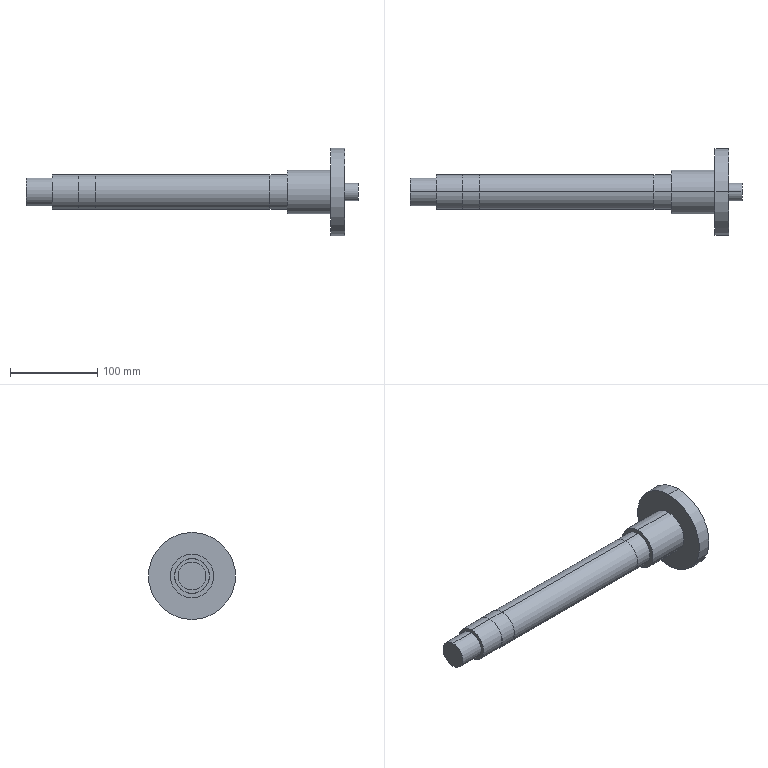Component | SolidWorks | Axis-1 | 1 solid | 25 faces | box 381 x 100 x 100 mm | volume 589087 mm3 | cylinder 16 | plane 9 | commonest cylinder face diameters 39.8 x4 40 x4 20 x2 32 x2 100 x2 50 x2
build123d program:
from build123d import *

# Parameters (mm, degrees)
SKETCH2_OUTSIDE_W   = 180.474
SKETCH2_OUTSIDE_H   = 180.474
SKETCH2_OUTSIDE_R   = 19.9
CUT_EXTRUDE1_DEPTH  = 30
SKETCH3_R           = 10
BOSS_EXTRUDE1_DEPTH = 15


with BuildPart() as part:
    # Sketch1 → Revolve1 (revolve)
    with BuildSketch(Plane.XY, mode=Mode.PRIVATE) as revolve1_sk:
        Polygon((0, 0), (0, 16), (30, 16), (30, 20), (80, 20), (80, 19.9), (280, 19.9), (280, 20), (300, 20), (300, 25), (350, 25), (350, 50), (366, 50), (366, 0), align=None)
    revolve(revolve1_sk.sketch.rotate(Axis((-164.625, 0, 0), (1, 0, 0)), 90), axis=Axis((-164.625, 0, 0), (1, 0, 0)))

    # Sketch2 outside → Cut-Extrude1 (cut)
    with BuildSketch(Plane.ZY.offset(-30)):
        Rectangle(SKETCH2_OUTSIDE_W, SKETCH2_OUTSIDE_H)
        Circle(SKETCH2_OUTSIDE_R, mode=Mode.SUBTRACT)
    extrude(amount=-CUT_EXTRUDE1_DEPTH, mode=Mode.SUBTRACT)

    # Sketch3 → Boss-Extrude1 (add)
    with BuildSketch(Plane(origin=(366, 0, 0), x_dir=(0, 0, -1), z_dir=(1, 0, 0))):
        with Locations(Location((0, 0, 0), (0, 0, 180))):
            Circle(SKETCH3_R)
    extrude(amount=BOSS_EXTRUDE1_DEPTH)


solid = part.part

# Placed as in the assembly
solid = solid.moved(Location((-372.743, 1299.706, 687.116), (0, 0, 0)))
STEP:
#1=COLOUR_RGB('',0.7922,0.8196,0.9333);
#2=FILL_AREA_STYLE_COLOUR('',#1);
#3=FILL_AREA_STYLE('',(#2));
#4=SURFACE_STYLE_FILL_AREA(#3);
#5=SURFACE_SIDE_STYLE('',(#4));
#6=SURFACE_STYLE_USAGE(.BOTH.,#5);
#7=PRESENTATION_STYLE_ASSIGNMENT((#6));
#8=CARTESIAN_POINT('',(0.3251,51.17,26.658));
#9=VERTEX_POINT('',#8);
#10=CARTESIAN_POINT('',(0.3251,51.17,27.446));
#11=VERTEX_POINT('',#10);
#12=CARTESIAN_POINT('',(0.3251,51.17,27.052));
#13=DIRECTION('',(1.,0.,0.));
#14=DIRECTION('',(0.,0.,-1.));
#15=AXIS2_PLACEMENT_3D('',#12,#13,#14);
#16=CIRCLE('',#15,0.3937);
#17=EDGE_CURVE('',#9,#11,#16,.T.);
#18=ORIENTED_EDGE('',*,*,#17,.F.);
#19=CARTESIAN_POINT('',(-0.2655,51.17,26.658));
#20=VERTEX_POINT('',#19);
#21=CARTESIAN_POINT('',(0.3251,51.17,26.658));
#22=DIRECTION('',(-1.,0.,0.));
#23=VECTOR('',#22,39.37);
#24=LINE('',#21,#23);
#25=EDGE_CURVE('',#9,#20,#24,.T.);
#26=ORIENTED_EDGE('',*,*,#25,.T.);
#27=CARTESIAN_POINT('',(-0.2655,51.17,27.446));
#28=VERTEX_POINT('',#27);
#29=CARTESIAN_POINT('',(-0.2655,51.17,27.052));
#30=DIRECTION('',(1.,0.,0.));
#31=DIRECTION('',(0.,0.,1.));
#32=AXIS2_PLACEMENT_3D('',#29,#30,#31);
#33=CIRCLE('',#32,0.3937);
#34=EDGE_CURVE('',#20,#28,#33,.T.);
#35=ORIENTED_EDGE('',*,*,#34,.T.);
#36=CARTESIAN_POINT('',(0.3251,51.17,27.446));
#37=DIRECTION('',(-1.,0.,0.));
#38=VECTOR('',#37,39.37);
#39=LINE('',#36,#38);
#40=EDGE_CURVE('',#11,#28,#39,.T.);
#41=ORIENTED_EDGE('',*,*,#40,.F.);
#42=EDGE_LOOP('',(#18,#26,#35,#41));
#43=FACE_OUTER_BOUND('',#42,.T.);
#44=CARTESIAN_POINT('',(0.3251,51.17,27.052));
#45=DIRECTION('',(-1.,0.,0.));
#46=DIRECTION('',(0.,0.,1.));
#47=AXIS2_PLACEMENT_3D('',#44,#45,#46);
#48=CYLINDRICAL_SURFACE('',#47,0.3937);
#49=ADVANCED_FACE('',(#43),#48,.T.);
#50=CARTESIAN_POINT('',(-13.494,51.17,27.682));
#51=VERTEX_POINT('',#50);
#52=CARTESIAN_POINT('',(-13.494,51.17,26.422));
#53=VERTEX_POINT('',#52);
#54=CARTESIAN_POINT('',(-13.494,51.17,27.052));
#55=DIRECTION('',(-1.,0.,0.));
#56=DIRECTION('',(0.,0.,1.));
#57=AXIS2_PLACEMENT_3D('',#54,#55,#56);
#58=CIRCLE('',#57,0.6299);
#59=EDGE_CURVE('',#51,#53,#58,.T.);
#60=ORIENTED_EDGE('',*,*,#59,.T.);
#61=CARTESIAN_POINT('',(-14.675,51.17,26.422));
#62=VERTEX_POINT('',#61);
#63=CARTESIAN_POINT('',(-21.156,51.17,26.422));
#64=DIRECTION('',(-1.,0.,0.));
#65=VECTOR('',#64,39.37);
#66=LINE('',#63,#65);
#67=EDGE_CURVE('',#53,#62,#66,.T.);
#68=ORIENTED_EDGE('',*,*,#67,.T.);
#69=CARTESIAN_POINT('',(-14.675,51.17,27.682));
#70=VERTEX_POINT('',#69);
#71=CARTESIAN_POINT('',(-14.675,51.17,27.052));
#72=DIRECTION('',(-1.,0.,0.));
#73=DIRECTION('',(0.,0.,1.));
#74=AXIS2_PLACEMENT_3D('',#71,#72,#73);
#75=CIRCLE('',#74,0.6299);
#76=EDGE_CURVE('',#70,#62,#75,.T.);
#77=ORIENTED_EDGE('',*,*,#76,.F.);
#78=CARTESIAN_POINT('',(-21.156,51.17,27.682));
#79=DIRECTION('',(-1.,0.,0.));
#80=VECTOR('',#79,39.37);
#81=LINE('',#78,#80);
#82=EDGE_CURVE('',#51,#70,#81,.T.);
#83=ORIENTED_EDGE('',*,*,#82,.F.);
#84=EDGE_LOOP('',(#60,#68,#77,#83));
#85=FACE_OUTER_BOUND('',#84,.T.);
#86=CARTESIAN_POINT('',(-21.156,51.17,27.052));
#87=DIRECTION('',(-1.,0.,0.));
#88=DIRECTION('',(0.,0.,1.));
#89=AXIS2_PLACEMENT_3D('',#86,#87,#88);
#90=CYLINDRICAL_SURFACE('',#89,0.6299);
#91=ADVANCED_FACE('',(#85),#90,.T.);
#92=CARTESIAN_POINT('',(-12.313,51.17,27.835));
#93=VERTEX_POINT('',#92);
#94=CARTESIAN_POINT('',(-12.313,51.17,26.268));
#95=VERTEX_POINT('',#94);
#96=CARTESIAN_POINT('',(-12.313,51.17,27.052));
#97=DIRECTION('',(-1.,0.,0.));
#98=DIRECTION('',(0.,0.,1.));
#99=AXIS2_PLACEMENT_3D('',#96,#97,#98);
#100=CIRCLE('',#99,0.7835);
#101=EDGE_CURVE('',#93,#95,#100,.T.);
#102=ORIENTED_EDGE('',*,*,#101,.T.);
#103=CARTESIAN_POINT('',(-13.494,51.17,26.268));
#104=VERTEX_POINT('',#103);
#105=CARTESIAN_POINT('',(-12.313,51.17,26.268));
#106=DIRECTION('',(-1.,0.,0.));
#107=VECTOR('',#106,39.37);
#108=LINE('',#105,#107);
#109=EDGE_CURVE('',#95,#104,#108,.T.);
#110=ORIENTED_EDGE('',*,*,#109,.T.);
#111=CARTESIAN_POINT('',(-13.494,51.17,27.835));
#112=VERTEX_POINT('',#111);
#113=CARTESIAN_POINT('',(-13.494,51.17,27.052));
#114=DIRECTION('',(-1.,0.,0.));
#115=DIRECTION('',(0.,0.,1.));
#116=AXIS2_PLACEMENT_3D('',#113,#114,#115);
#117=CIRCLE('',#116,0.7835);
#118=EDGE_CURVE('',#112,#104,#117,.T.);
#119=ORIENTED_EDGE('',*,*,#118,.F.);
#120=CARTESIAN_POINT('',(-12.313,51.17,27.835));
#121=DIRECTION('',(-1.,0.,0.));
#122=VECTOR('',#121,39.37);
#123=LINE('',#120,#122);
#124=EDGE_CURVE('',#93,#112,#123,.T.);
#125=ORIENTED_EDGE('',*,*,#124,.F.);
#126=EDGE_LOOP('',(#102,#110,#119,#125));
#127=FACE_OUTER_BOUND('',#126,.T.);
#128=CARTESIAN_POINT('',(-12.313,51.17,27.052));
#129=DIRECTION('',(-1.,0.,0.));
#130=DIRECTION('',(0.,0.,1.));
#131=AXIS2_PLACEMENT_3D('',#128,#129,#130);
#132=CYLINDRICAL_SURFACE('',#131,0.7835);
#133=ADVANCED_FACE('',(#127),#132,.T.);
#134=CARTESIAN_POINT('',(-0.2655,51.17,29.02));
#135=VERTEX_POINT('',#134);
#136=CARTESIAN_POINT('',(-0.2655,51.17,25.083));
#137=VERTEX_POINT('',#136);
#138=CARTESIAN_POINT('',(-0.2655,51.17,27.052));
#139=DIRECTION('',(-1.,0.,0.));
#140=DIRECTION('',(0.,0.,1.));
#141=AXIS2_PLACEMENT_3D('',#138,#139,#140);
#142=CIRCLE('',#141,1.969);
#143=EDGE_CURVE('',#135,#137,#142,.T.);
#144=ORIENTED_EDGE('',*,*,#143,.T.);
#145=CARTESIAN_POINT('',(-0.8954,51.17,25.083));
#146=VERTEX_POINT('',#145);
#147=CARTESIAN_POINT('',(-21.156,51.17,25.083));
#148=DIRECTION('',(-1.,0.,0.));
#149=VECTOR('',#148,39.37);
#150=LINE('',#147,#149);
#151=EDGE_CURVE('',#137,#146,#150,.T.);
#152=ORIENTED_EDGE('',*,*,#151,.T.);
#153=CARTESIAN_POINT('',(-0.8954,51.17,29.02));
#154=VERTEX_POINT('',#153);
#155=CARTESIAN_POINT('',(-0.8954,51.17,27.052));
#156=DIRECTION('',(-1.,0.,0.));
#157=DIRECTION('',(0.,0.,1.));
#158=AXIS2_PLACEMENT_3D('',#155,#156,#157);
#159=CIRCLE('',#158,1.969);
#160=EDGE_CURVE('',#154,#146,#159,.T.);
#161=ORIENTED_EDGE('',*,*,#160,.F.);
#162=CARTESIAN_POINT('',(-21.156,51.17,29.02));
#163=DIRECTION('',(-1.,0.,0.));
#164=VECTOR('',#163,39.37);
#165=LINE('',#162,#164);
#166=EDGE_CURVE('',#135,#154,#165,.T.);
#167=ORIENTED_EDGE('',*,*,#166,.F.);
#168=EDGE_LOOP('',(#144,#152,#161,#167));
#169=FACE_OUTER_BOUND('',#168,.T.);
#170=CARTESIAN_POINT('',(-21.156,51.17,27.052));
#171=DIRECTION('',(-1.,0.,0.));
#172=DIRECTION('',(0.,0.,1.));
#173=AXIS2_PLACEMENT_3D('',#170,#171,#172);
#174=CYLINDRICAL_SURFACE('',#173,1.969);
#175=ADVANCED_FACE('',(#169),#174,.T.);
#176=CARTESIAN_POINT('',(-0.8954,51.17,28.036));
#177=VERTEX_POINT('',#176);
#178=CARTESIAN_POINT('',(-0.8954,51.17,26.068));
#179=VERTEX_POINT('',#178);
#180=CARTESIAN_POINT('',(-0.8954,51.17,27.052));
#181=DIRECTION('',(-1.,0.,0.));
#182=DIRECTION('',(0.,0.,1.));
#183=AXIS2_PLACEMENT_3D('',#180,#181,#182);
#184=CIRCLE('',#183,0.9843);
#185=EDGE_CURVE('',#177,#179,#184,.T.);
#186=ORIENTED_EDGE('',*,*,#185,.T.);
#187=CARTESIAN_POINT('',(-2.864,51.17,26.068));
#188=VERTEX_POINT('',#187);
#189=CARTESIAN_POINT('',(-21.156,51.17,26.068));
#190=DIRECTION('',(-1.,0.,0.));
#191=VECTOR('',#190,39.37);
#192=LINE('',#189,#191);
#193=EDGE_CURVE('',#179,#188,#192,.T.);
#194=ORIENTED_EDGE('',*,*,#193,.T.);
#195=CARTESIAN_POINT('',(-2.864,51.17,28.036));
#196=VERTEX_POINT('',#195);
#197=CARTESIAN_POINT('',(-2.864,51.17,27.052));
#198=DIRECTION('',(-1.,0.,0.));
#199=DIRECTION('',(0.,0.,1.));
#200=AXIS2_PLACEMENT_3D('',#197,#198,#199);
#201=CIRCLE('',#200,0.9843);
#202=EDGE_CURVE('',#196,#188,#201,.T.);
#203=ORIENTED_EDGE('',*,*,#202,.F.);
#204=CARTESIAN_POINT('',(-21.156,51.17,28.036));
#205=DIRECTION('',(-1.,0.,0.));
#206=VECTOR('',#205,39.37);
#207=LINE('',#204,#206);
#208=EDGE_CURVE('',#177,#196,#207,.T.);
#209=ORIENTED_EDGE('',*,*,#208,.F.);
#210=EDGE_LOOP('',(#186,#194,#203,#209));
#211=FACE_OUTER_BOUND('',#210,.T.);
#212=CARTESIAN_POINT('',(-21.156,51.17,27.052));
#213=DIRECTION('',(-1.,0.,0.));
#214=DIRECTION('',(0.,0.,1.));
#215=AXIS2_PLACEMENT_3D('',#212,#213,#214);
#216=CYLINDRICAL_SURFACE('',#215,0.9843);
#217=ADVANCED_FACE('',(#211),#216,.T.);
#218=CARTESIAN_POINT('',(-2.864,51.17,27.839));
#219=VERTEX_POINT('',#218);
#220=CARTESIAN_POINT('',(-2.864,51.17,26.264));
#221=VERTEX_POINT('',#220);
#222=CARTESIAN_POINT('',(-2.864,51.17,27.052));
#223=DIRECTION('',(-1.,0.,0.));
#224=DIRECTION('',(0.,0.,1.));
#225=AXIS2_PLACEMENT_3D('',#222,#223,#224);
#226=CIRCLE('',#225,0.7874);
#227=EDGE_CURVE('',#219,#221,#226,.T.);
#228=ORIENTED_EDGE('',*,*,#227,.T.);
#229=CARTESIAN_POINT('',(-3.651,51.17,26.264));
#230=VERTEX_POINT('',#229);
#231=CARTESIAN_POINT('',(-21.156,51.17,26.264));
#232=DIRECTION('',(-1.,0.,0.));
#233=VECTOR('',#232,39.37);
#234=LINE('',#231,#233);
#235=EDGE_CURVE('',#221,#230,#234,.T.);
#236=ORIENTED_EDGE('',*,*,#235,.T.);
#237=CARTESIAN_POINT('',(-3.651,51.17,27.839));
#238=VERTEX_POINT('',#237);
#239=CARTESIAN_POINT('',(-3.651,51.17,27.052));
#240=DIRECTION('',(-1.,0.,0.));
#241=DIRECTION('',(0.,0.,1.));
#242=AXIS2_PLACEMENT_3D('',#239,#240,#241);
#243=CIRCLE('',#242,0.7874);
#244=EDGE_CURVE('',#238,#230,#243,.T.);
#245=ORIENTED_EDGE('',*,*,#244,.F.);
#246=CARTESIAN_POINT('',(-21.156,51.17,27.839));
#247=DIRECTION('',(-1.,0.,0.));
#248=VECTOR('',#247,39.37);
#249=LINE('',#246,#248);
#250=EDGE_CURVE('',#219,#238,#249,.T.);
#251=ORIENTED_EDGE('',*,*,#250,.F.);
#252=EDGE_LOOP('',(#228,#236,#245,#251));
#253=FACE_OUTER_BOUND('',#252,.T.);
#254=CARTESIAN_POINT('',(-21.156,51.17,27.052));
#255=DIRECTION('',(-1.,0.,0.));
#256=DIRECTION('',(0.,0.,1.));
#257=AXIS2_PLACEMENT_3D('',#254,#255,#256);
#258=CYLINDRICAL_SURFACE('',#257,0.7874);
#259=ADVANCED_FACE('',(#253),#258,.T.);
#260=CARTESIAN_POINT('',(-3.651,51.17,27.835));
#261=VERTEX_POINT('',#260);
#262=CARTESIAN_POINT('',(-3.651,51.17,26.268));
#263=VERTEX_POINT('',#262);
#264=CARTESIAN_POINT('',(-3.651,51.17,27.052));
#265=DIRECTION('',(-1.,0.,0.));
#266=DIRECTION('',(0.,0.,1.));
#267=AXIS2_PLACEMENT_3D('',#264,#265,#266);
#268=CIRCLE('',#267,0.7835);
#269=EDGE_CURVE('',#261,#263,#268,.T.);
#270=ORIENTED_EDGE('',*,*,#269,.T.);
#271=CARTESIAN_POINT('',(-11.525,51.17,26.268));
#272=VERTEX_POINT('',#271);
#273=CARTESIAN_POINT('',(-21.156,51.17,26.268));
#274=DIRECTION('',(-1.,0.,0.));
#275=VECTOR('',#274,39.37);
#276=LINE('',#273,#275);
#277=EDGE_CURVE('',#263,#272,#276,.T.);
#278=ORIENTED_EDGE('',*,*,#277,.T.);
#279=CARTESIAN_POINT('',(-11.525,51.17,27.835));
#280=VERTEX_POINT('',#279);
#281=CARTESIAN_POINT('',(-11.525,51.17,27.052));
#282=DIRECTION('',(-1.,0.,0.));
#283=DIRECTION('',(0.,0.,1.));
#284=AXIS2_PLACEMENT_3D('',#281,#282,#283);
#285=CIRCLE('',#284,0.7835);
#286=EDGE_CURVE('',#280,#272,#285,.T.);
#287=ORIENTED_EDGE('',*,*,#286,.F.);
#288=CARTESIAN_POINT('',(-21.156,51.17,27.835));
#289=DIRECTION('',(-1.,0.,0.));
#290=VECTOR('',#289,39.37);
#291=LINE('',#288,#290);
#292=EDGE_CURVE('',#261,#280,#291,.T.);
#293=ORIENTED_EDGE('',*,*,#292,.F.);
#294=EDGE_LOOP('',(#270,#278,#287,#293));
#295=FACE_OUTER_BOUND('',#294,.T.);
#296=CARTESIAN_POINT('',(-21.156,51.17,27.052));
#297=DIRECTION('',(-1.,0.,0.));
#298=DIRECTION('',(0.,0.,1.));
#299=AXIS2_PLACEMENT_3D('',#296,#297,#298);
#300=CYLINDRICAL_SURFACE('',#299,0.7835);
#301=ADVANCED_FACE('',(#295),#300,.T.);
#302=CARTESIAN_POINT('',(-11.525,51.17,27.839));
#303=VERTEX_POINT('',#302);
#304=CARTESIAN_POINT('',(-11.525,51.17,26.264));
#305=VERTEX_POINT('',#304);
#306=CARTESIAN_POINT('',(-11.525,51.17,27.052));
#307=DIRECTION('',(-1.,0.,0.));
#308=DIRECTION('',(0.,0.,1.));
#309=AXIS2_PLACEMENT_3D('',#306,#307,#308);
#310=CIRCLE('',#309,0.7874);
#311=EDGE_CURVE('',#303,#305,#310,.T.);
#312=ORIENTED_EDGE('',*,*,#311,.T.);
#313=CARTESIAN_POINT('',(-12.313,51.17,26.264));
#314=VERTEX_POINT('',#313);
#315=CARTESIAN_POINT('',(-21.156,51.17,26.264));
#316=DIRECTION('',(-1.,0.,0.));
#317=VECTOR('',#316,39.37);
#318=LINE('',#315,#317);
#319=EDGE_CURVE('',#305,#314,#318,.T.);
#320=ORIENTED_EDGE('',*,*,#319,.T.);
#321=CARTESIAN_POINT('',(-12.313,51.17,27.839));
#322=VERTEX_POINT('',#321);
#323=CARTESIAN_POINT('',(-12.313,51.17,27.052));
#324=DIRECTION('',(-1.,0.,0.));
#325=DIRECTION('',(0.,0.,1.));
#326=AXIS2_PLACEMENT_3D('',#323,#324,#325);
#327=CIRCLE('',#326,0.7874);
#328=EDGE_CURVE('',#322,#314,#327,.T.);
#329=ORIENTED_EDGE('',*,*,#328,.F.);
#330=CARTESIAN_POINT('',(-21.156,51.17,27.839));
#331=DIRECTION('',(-1.,0.,0.));
#332=VECTOR('',#331,39.37);
#333=LINE('',#330,#332);
#334=EDGE_CURVE('',#303,#322,#333,.T.);
#335=ORIENTED_EDGE('',*,*,#334,.F.);
#336=EDGE_LOOP('',(#312,#320,#329,#335));
#337=FACE_OUTER_BOUND('',#336,.T.);
#338=CARTESIAN_POINT('',(-21.156,51.17,27.052));
#339=DIRECTION('',(-1.,0.,0.));
#340=DIRECTION('',(0.,0.,1.));
#341=AXIS2_PLACEMENT_3D('',#338,#339,#340);
#342=CYLINDRICAL_SURFACE('',#341,0.7874);
#343=ADVANCED_FACE('',(#337),#342,.T.);
#344=ORIENTED_EDGE('',*,*,#319,.F.);
#345=CARTESIAN_POINT('',(-11.525,51.17,27.052));
#346=DIRECTION('',(-1.,0.,0.));
#347=DIRECTION('',(0.,0.,1.));
#348=AXIS2_PLACEMENT_3D('',#345,#346,#347);
#349=CIRCLE('',#348,0.7874);
#350=EDGE_CURVE('',#305,#303,#349,.T.);
#351=ORIENTED_EDGE('',*,*,#350,.T.);
#352=ORIENTED_EDGE('',*,*,#334,.T.);
#353=CARTESIAN_POINT('',(-12.313,51.17,27.052));
#354=DIRECTION('',(-1.,0.,0.));
#355=DIRECTION('',(0.,0.,1.));
#356=AXIS2_PLACEMENT_3D('',#353,#354,#355);
#357=CIRCLE('',#356,0.7874);
#358=EDGE_CURVE('',#314,#322,#357,.T.);
#359=ORIENTED_EDGE('',*,*,#358,.F.);
#360=EDGE_LOOP('',(#344,#351,#352,#359));
#361=FACE_OUTER_BOUND('',#360,.T.);
#362=CARTESIAN_POINT('',(-21.156,51.17,27.052));
#363=DIRECTION('',(-1.,0.,0.));
#364=DIRECTION('',(0.,0.,1.));
#365=AXIS2_PLACEMENT_3D('',#362,#363,#364);
#366=CYLINDRICAL_SURFACE('',#365,0.7874);
#367=ADVANCED_FACE('',(#361),#366,.T.);
#368=ORIENTED_EDGE('',*,*,#311,.F.);
#369=ORIENTED_EDGE('',*,*,#350,.F.);
#370=EDGE_LOOP('',(#368,#369));
#371=FACE_OUTER_BOUND('',#370,.T.);
#372=ORIENTED_EDGE('',*,*,#286,.T.);
#373=CARTESIAN_POINT('',(-11.525,51.17,27.052));
#374=DIRECTION('',(-1.,0.,0.));
#375=DIRECTION('',(0.,0.,1.));
#376=AXIS2_PLACEMENT_3D('',#373,#374,#375);
#377=CIRCLE('',#376,0.7835);
#378=EDGE_CURVE('',#272,#280,#377,.T.);
#379=ORIENTED_EDGE('',*,*,#378,.T.);
#380=EDGE_LOOP('',(#372,#379));
#381=FACE_BOUND('',#380,.T.);
#382=CARTESIAN_POINT('',(-11.525,51.957,27.052));
#383=DIRECTION('',(-1.,0.,0.));
#384=DIRECTION('',(0.,0.,1.));
#385=AXIS2_PLACEMENT_3D('',#382,#383,#384);
#386=PLANE('',#385);
#387=ADVANCED_FACE('',(#371,#381),#386,.F.);
#388=ORIENTED_EDGE('',*,*,#277,.F.);
#389=CARTESIAN_POINT('',(-3.651,51.17,27.052));
#390=DIRECTION('',(-1.,0.,0.));
#391=DIRECTION('',(0.,0.,1.));
#392=AXIS2_PLACEMENT_3D('',#389,#390,#391);
#393=CIRCLE('',#392,0.7835);
#394=EDGE_CURVE('',#263,#261,#393,.T.);
#395=ORIENTED_EDGE('',*,*,#394,.T.);
#396=ORIENTED_EDGE('',*,*,#292,.T.);
#397=ORIENTED_EDGE('',*,*,#378,.F.);
#398=EDGE_LOOP('',(#388,#395,#396,#397));
#399=FACE_OUTER_BOUND('',#398,.T.);
#400=CARTESIAN_POINT('',(-21.156,51.17,27.052));
#401=DIRECTION('',(-1.,0.,0.));
#402=DIRECTION('',(0.,0.,1.));
#403=AXIS2_PLACEMENT_3D('',#400,#401,#402);
#404=CYLINDRICAL_SURFACE('',#403,0.7835);
#405=ADVANCED_FACE('',(#399),#404,.T.);
#406=ORIENTED_EDGE('',*,*,#269,.F.);
#407=ORIENTED_EDGE('',*,*,#394,.F.);
#408=EDGE_LOOP('',(#406,#407));
#409=FACE_BOUND('',#408,.T.);
#410=ORIENTED_EDGE('',*,*,#244,.T.);
#411=CARTESIAN_POINT('',(-3.651,51.17,27.052));
#412=DIRECTION('',(-1.,0.,0.));
#413=DIRECTION('',(0.,0.,1.));
#414=AXIS2_PLACEMENT_3D('',#411,#412,#413);
#415=CIRCLE('',#414,0.7874);
#416=EDGE_CURVE('',#230,#238,#415,.T.);
#417=ORIENTED_EDGE('',*,*,#416,.T.);
#418=EDGE_LOOP('',(#410,#417));
#419=FACE_OUTER_BOUND('',#418,.T.);
#420=CARTESIAN_POINT('',(-3.651,51.953,27.052));
#421=DIRECTION('',(1.,0.,0.));
#422=DIRECTION('',(0.,0.,-1.));
#423=AXIS2_PLACEMENT_3D('',#420,#421,#422);
#424=PLANE('',#423);
#425=ADVANCED_FACE('',(#409,#419),#424,.F.);
#426=ORIENTED_EDGE('',*,*,#235,.F.);
#427=CARTESIAN_POINT('',(-2.864,51.17,27.052));
#428=DIRECTION('',(-1.,0.,0.));
#429=DIRECTION('',(0.,0.,1.));
#430=AXIS2_PLACEMENT_3D('',#427,#428,#429);
#431=CIRCLE('',#430,0.7874);
#432=EDGE_CURVE('',#221,#219,#431,.T.);
#433=ORIENTED_EDGE('',*,*,#432,.T.);
#434=ORIENTED_EDGE('',*,*,#250,.T.);
#435=ORIENTED_EDGE('',*,*,#416,.F.);
#436=EDGE_LOOP('',(#426,#433,#434,#435));
#437=FACE_OUTER_BOUND('',#436,.T.);
#438=CARTESIAN_POINT('',(-21.156,51.17,27.052));
#439=DIRECTION('',(-1.,0.,0.));
#440=DIRECTION('',(0.,0.,1.));
#441=AXIS2_PLACEMENT_3D('',#438,#439,#440);
#442=CYLINDRICAL_SURFACE('',#441,0.7874);
#443=ADVANCED_FACE('',(#437),#442,.T.);
#444=ORIENTED_EDGE('',*,*,#227,.F.);
#445=ORIENTED_EDGE('',*,*,#432,.F.);
#446=EDGE_LOOP('',(#444,#445));
#447=FACE_BOUND('',#446,.T.);
#448=ORIENTED_EDGE('',*,*,#202,.T.);
#449=CARTESIAN_POINT('',(-2.864,51.17,27.052));
#450=DIRECTION('',(-1.,0.,0.));
#451=DIRECTION('',(0.,0.,1.));
#452=AXIS2_PLACEMENT_3D('',#449,#450,#451);
#453=CIRCLE('',#452,0.9843);
#454=EDGE_CURVE('',#188,#196,#453,.T.);
#455=ORIENTED_EDGE('',*,*,#454,.T.);
#456=EDGE_LOOP('',(#448,#455));
#457=FACE_OUTER_BOUND('',#456,.T.);
#458=CARTESIAN_POINT('',(-2.864,51.957,27.052));
#459=DIRECTION('',(1.,0.,0.));
#460=DIRECTION('',(0.,0.,-1.));
#461=AXIS2_PLACEMENT_3D('',#458,#459,#460);
#462=PLANE('',#461);
#463=ADVANCED_FACE('',(#447,#457),#462,.F.);
#464=ORIENTED_EDGE('',*,*,#193,.F.);
#465=CARTESIAN_POINT('',(-0.8954,51.17,27.052));
#466=DIRECTION('',(-1.,0.,0.));
#467=DIRECTION('',(0.,0.,1.));
#468=AXIS2_PLACEMENT_3D('',#465,#466,#467);
#469=CIRCLE('',#468,0.9843);
#470=EDGE_CURVE('',#179,#177,#469,.T.);
#471=ORIENTED_EDGE('',*,*,#470,.T.);
#472=ORIENTED_EDGE('',*,*,#208,.T.);
#473=ORIENTED_EDGE('',*,*,#454,.F.);
#474=EDGE_LOOP('',(#464,#471,#472,#473));
#475=FACE_OUTER_BOUND('',#474,.T.);
#476=CARTESIAN_POINT('',(-21.156,51.17,27.052));
#477=DIRECTION('',(-1.,0.,0.));
#478=DIRECTION('',(0.,0.,1.));
#479=AXIS2_PLACEMENT_3D('',#476,#477,#478);
#480=CYLINDRICAL_SURFACE('',#479,0.9843);
#481=ADVANCED_FACE('',(#475),#480,.T.);
#482=ORIENTED_EDGE('',*,*,#185,.F.);
#483=ORIENTED_EDGE('',*,*,#470,.F.);
#484=EDGE_LOOP('',(#482,#483));
#485=FACE_BOUND('',#484,.T.);
#486=ORIENTED_EDGE('',*,*,#160,.T.);
#487=CARTESIAN_POINT('',(-0.8954,51.17,27.052));
#488=DIRECTION('',(-1.,0.,0.));
#489=DIRECTION('',(0.,0.,1.));
#490=AXIS2_PLACEMENT_3D('',#487,#488,#489);
#491=CIRCLE('',#490,1.969);
#492=EDGE_CURVE('',#146,#154,#491,.T.);
#493=ORIENTED_EDGE('',*,*,#492,.T.);
#494=EDGE_LOOP('',(#486,#493));
#495=FACE_OUTER_BOUND('',#494,.T.);
#496=CARTESIAN_POINT('',(-0.8954,52.154,27.052));
#497=DIRECTION('',(1.,0.,0.));
#498=DIRECTION('',(0.,0.,-1.));
#499=AXIS2_PLACEMENT_3D('',#496,#497,#498);
#500=PLANE('',#499);
#501=ADVANCED_FACE('',(#485,#495),#500,.F.);
#502=ORIENTED_EDGE('',*,*,#151,.F.);
#503=CARTESIAN_POINT('',(-0.2655,51.17,27.052));
#504=DIRECTION('',(-1.,0.,0.));
#505=DIRECTION('',(0.,0.,1.));
#506=AXIS2_PLACEMENT_3D('',#503,#504,#505);
#507=CIRCLE('',#506,1.969);
#508=EDGE_CURVE('',#137,#135,#507,.T.);
#509=ORIENTED_EDGE('',*,*,#508,.T.);
#510=ORIENTED_EDGE('',*,*,#166,.T.);
#511=ORIENTED_EDGE('',*,*,#492,.F.);
#512=EDGE_LOOP('',(#502,#509,#510,#511));
#513=FACE_OUTER_BOUND('',#512,.T.);
#514=CARTESIAN_POINT('',(-21.156,51.17,27.052));
#515=DIRECTION('',(-1.,0.,0.));
#516=DIRECTION('',(0.,0.,1.));
#517=AXIS2_PLACEMENT_3D('',#514,#515,#516);
#518=CYLINDRICAL_SURFACE('',#517,1.969);
#519=ADVANCED_FACE('',(#513),#518,.T.);
#520=CARTESIAN_POINT('',(-0.2655,51.17,27.052));
#521=DIRECTION('',(1.,0.,0.));
#522=DIRECTION('',(0.,0.,1.));
#523=AXIS2_PLACEMENT_3D('',#520,#521,#522);
#524=CIRCLE('',#523,0.3937);
#525=EDGE_CURVE('',#28,#20,#524,.T.);
#526=ORIENTED_EDGE('',*,*,#525,.F.);
#527=ORIENTED_EDGE('',*,*,#34,.F.);
#528=EDGE_LOOP('',(#526,#527));
#529=FACE_BOUND('',#528,.T.);
#530=ORIENTED_EDGE('',*,*,#143,.F.);
#531=ORIENTED_EDGE('',*,*,#508,.F.);
#532=EDGE_LOOP('',(#530,#531));
#533=FACE_OUTER_BOUND('',#532,.T.);
#534=CARTESIAN_POINT('',(-0.2655,53.138,27.052));
#535=DIRECTION('',(-1.,0.,0.));
#536=DIRECTION('',(0.,0.,1.));
#537=AXIS2_PLACEMENT_3D('',#534,#535,#536);
#538=PLANE('',#537);
#539=ADVANCED_FACE('',(#529,#533),#538,.F.);
#540=ORIENTED_EDGE('',*,*,#101,.F.);
#541=CARTESIAN_POINT('',(-12.313,51.17,27.052));
#542=DIRECTION('',(-1.,0.,0.));
#543=DIRECTION('',(0.,0.,1.));
#544=AXIS2_PLACEMENT_3D('',#541,#542,#543);
#545=CIRCLE('',#544,0.7835);
#546=EDGE_CURVE('',#95,#93,#545,.T.);
#547=ORIENTED_EDGE('',*,*,#546,.F.);
#548=EDGE_LOOP('',(#540,#547));
#549=FACE_BOUND('',#548,.T.);
#550=ORIENTED_EDGE('',*,*,#328,.T.);
#551=ORIENTED_EDGE('',*,*,#358,.T.);
#552=EDGE_LOOP('',(#550,#551));
#553=FACE_OUTER_BOUND('',#552,.T.);
#554=CARTESIAN_POINT('',(-12.313,51.17,27.052));
#555=DIRECTION('',(-1.,0.,0.));
#556=DIRECTION('',(0.,0.,1.));
#557=AXIS2_PLACEMENT_3D('',#554,#555,#556);
#558=PLANE('',#557);
#559=ADVANCED_FACE('',(#549,#553),#558,.T.);
#560=ORIENTED_EDGE('',*,*,#109,.F.);
#561=ORIENTED_EDGE('',*,*,#546,.T.);
#562=ORIENTED_EDGE('',*,*,#124,.T.);
#563=CARTESIAN_POINT('',(-13.494,51.17,27.052));
#564=DIRECTION('',(-1.,0.,0.));
#565=DIRECTION('',(0.,0.,1.));
#566=AXIS2_PLACEMENT_3D('',#563,#564,#565);
#567=CIRCLE('',#566,0.7835);
#568=EDGE_CURVE('',#104,#112,#567,.T.);
#569=ORIENTED_EDGE('',*,*,#568,.F.);
#570=EDGE_LOOP('',(#560,#561,#562,#569));
#571=FACE_OUTER_BOUND('',#570,.T.);
#572=CARTESIAN_POINT('',(-12.313,51.17,27.052));
#573=DIRECTION('',(-1.,0.,0.));
#574=DIRECTION('',(0.,0.,1.));
#575=AXIS2_PLACEMENT_3D('',#572,#573,#574);
#576=CYLINDRICAL_SURFACE('',#575,0.7835);
#577=ADVANCED_FACE('',(#571),#576,.T.);
#578=ORIENTED_EDGE('',*,*,#76,.T.);
#579=CARTESIAN_POINT('',(-14.675,51.17,27.052));
#580=DIRECTION('',(-1.,0.,0.));
#581=DIRECTION('',(0.,0.,1.));
#582=AXIS2_PLACEMENT_3D('',#579,#580,#581);
#583=CIRCLE('',#582,0.6299);
#584=EDGE_CURVE('',#62,#70,#583,.T.);
#585=ORIENTED_EDGE('',*,*,#584,.T.);
#586=EDGE_LOOP('',(#578,#585));
#587=FACE_OUTER_BOUND('',#586,.T.);
#588=CARTESIAN_POINT('',(-14.675,51.17,27.052));
#589=DIRECTION('',(1.,0.,0.));
#590=DIRECTION('',(0.,0.,-1.));
#591=AXIS2_PLACEMENT_3D('',#588,#589,#590);
#592=PLANE('',#591);
#593=ADVANCED_FACE('',(#587),#592,.F.);
#594=ORIENTED_EDGE('',*,*,#67,.F.);
#595=CARTESIAN_POINT('',(-13.494,51.17,27.052));
#596=DIRECTION('',(-1.,0.,0.));
#597=DIRECTION('',(0.,0.,1.));
#598=AXIS2_PLACEMENT_3D('',#595,#596,#597);
#599=CIRCLE('',#598,0.6299);
#600=EDGE_CURVE('',#53,#51,#599,.T.);
#601=ORIENTED_EDGE('',*,*,#600,.T.);
#602=ORIENTED_EDGE('',*,*,#82,.T.);
#603=ORIENTED_EDGE('',*,*,#584,.F.);
#604=EDGE_LOOP('',(#594,#601,#602,#603));
#605=FACE_OUTER_BOUND('',#604,.T.);
#606=CARTESIAN_POINT('',(-21.156,51.17,27.052));
#607=DIRECTION('',(-1.,0.,0.));
#608=DIRECTION('',(0.,0.,1.));
#609=AXIS2_PLACEMENT_3D('',#606,#607,#608);
#610=CYLINDRICAL_SURFACE('',#609,0.6299);
#611=ADVANCED_FACE('',(#605),#610,.T.);
#612=ORIENTED_EDGE('',*,*,#59,.F.);
#613=ORIENTED_EDGE('',*,*,#600,.F.);
#614=EDGE_LOOP('',(#612,#613));
#615=FACE_BOUND('',#614,.T.);
#616=ORIENTED_EDGE('',*,*,#118,.T.);
#617=ORIENTED_EDGE('',*,*,#568,.T.);
#618=EDGE_LOOP('',(#616,#617));
#619=FACE_OUTER_BOUND('',#618,.T.);
#620=CARTESIAN_POINT('',(-13.494,51.799,27.052));
#621=DIRECTION('',(1.,0.,0.));
#622=DIRECTION('',(0.,0.,-1.));
#623=AXIS2_PLACEMENT_3D('',#620,#621,#622);
#624=PLANE('',#623);
#625=ADVANCED_FACE('',(#615,#619),#624,.F.);
#626=ORIENTED_EDGE('',*,*,#25,.F.);
#627=CARTESIAN_POINT('',(0.3251,51.17,27.052));
#628=DIRECTION('',(1.,0.,0.));
#629=DIRECTION('',(0.,0.,-1.));
#630=AXIS2_PLACEMENT_3D('',#627,#628,#629);
#631=CIRCLE('',#630,0.3937);
#632=EDGE_CURVE('',#11,#9,#631,.T.);
#633=ORIENTED_EDGE('',*,*,#632,.F.);
#634=ORIENTED_EDGE('',*,*,#40,.T.);
#635=ORIENTED_EDGE('',*,*,#525,.T.);
#636=EDGE_LOOP('',(#626,#633,#634,#635));
#637=FACE_OUTER_BOUND('',#636,.T.);
#638=CARTESIAN_POINT('',(0.3251,51.17,27.052));
#639=DIRECTION('',(-1.,0.,0.));
#640=DIRECTION('',(0.,0.,1.));
#641=AXIS2_PLACEMENT_3D('',#638,#639,#640);
#642=CYLINDRICAL_SURFACE('',#641,0.3937);
#643=ADVANCED_FACE('',(#637),#642,.T.);
#644=ORIENTED_EDGE('',*,*,#632,.T.);
#645=ORIENTED_EDGE('',*,*,#17,.T.);
#646=EDGE_LOOP('',(#644,#645));
#647=FACE_OUTER_BOUND('',#646,.T.);
#648=CARTESIAN_POINT('',(0.3251,51.17,27.052));
#649=DIRECTION('',(1.,0.,0.));
#650=DIRECTION('',(0.,0.,-1.));
#651=AXIS2_PLACEMENT_3D('',#648,#649,#650);
#652=PLANE('',#651);
#653=ADVANCED_FACE('',(#647),#652,.T.);
#654=CLOSED_SHELL('',(#49,#91,#133,#175,#217,#259,#301,#343,#367,#387,#405,#425,#443,#463,#481,#501,#519,#539,#559,#577,#593,#611,#625,#643,#653));
#655=MANIFOLD_SOLID_BREP('',#654);
#656=STYLED_ITEM('',(#7),#655);
#657=(LENGTH_UNIT()NAMED_UNIT(*)SI_UNIT($,.METRE.));
#658=LENGTH_MEASURE_WITH_UNIT(LENGTH_MEASURE(0.0254),#657);
#659=DIMENSIONAL_EXPONENTS(1.,0.,0.,0.,0.,0.,0.);
#660=(CONVERSION_BASED_UNIT('',#658)LENGTH_UNIT()NAMED_UNIT(#659));
#661=UNCERTAINTY_MEASURE_WITH_UNIT(LENGTH_MEASURE(0.00001),#660,'','');
#662=(NAMED_UNIT(*)PLANE_ANGLE_UNIT()SI_UNIT($,.RADIAN.));
#663=(NAMED_UNIT(*)SI_UNIT($,.STERADIAN.)SOLID_ANGLE_UNIT());
#664=(GEOMETRIC_REPRESENTATION_CONTEXT(3)GLOBAL_UNCERTAINTY_ASSIGNED_CONTEXT((#661))GLOBAL_UNIT_ASSIGNED_CONTEXT((#660,#662,#663))REPRESENTATION_CONTEXT('',''));
#665=MECHANICAL_DESIGN_GEOMETRIC_PRESENTATION_REPRESENTATION('',(#656),#664);
#666=CARTESIAN_POINT('',(0.,0.,0.));
#667=DIRECTION('',(0.,0.,1.));
#668=DIRECTION('',(1.,0.,0.));
#669=AXIS2_PLACEMENT_3D('',#666,#667,#668);
#670=(LENGTH_UNIT()NAMED_UNIT(*)SI_UNIT($,.METRE.));
#671=LENGTH_MEASURE_WITH_UNIT(LENGTH_MEASURE(0.0254),#670);
#672=DIMENSIONAL_EXPONENTS(1.,0.,0.,0.,0.,0.,0.);
#673=(CONVERSION_BASED_UNIT('',#671)LENGTH_UNIT()NAMED_UNIT(#672));
#674=UNCERTAINTY_MEASURE_WITH_UNIT(LENGTH_MEASURE(0.00001),#673,'','');
#675=(NAMED_UNIT(*)PLANE_ANGLE_UNIT()SI_UNIT($,.RADIAN.));
#676=(NAMED_UNIT(*)SI_UNIT($,.STERADIAN.)SOLID_ANGLE_UNIT());
#677=(GEOMETRIC_REPRESENTATION_CONTEXT(3)GLOBAL_UNCERTAINTY_ASSIGNED_CONTEXT((#674))GLOBAL_UNIT_ASSIGNED_CONTEXT((#673,#675,#676))REPRESENTATION_CONTEXT('',''));
#678=ADVANCED_BREP_SHAPE_REPRESENTATION('',(#655,#669),#677);
#679=PRESENTATION_LAYER_ASSIGNMENT('','',(#656));